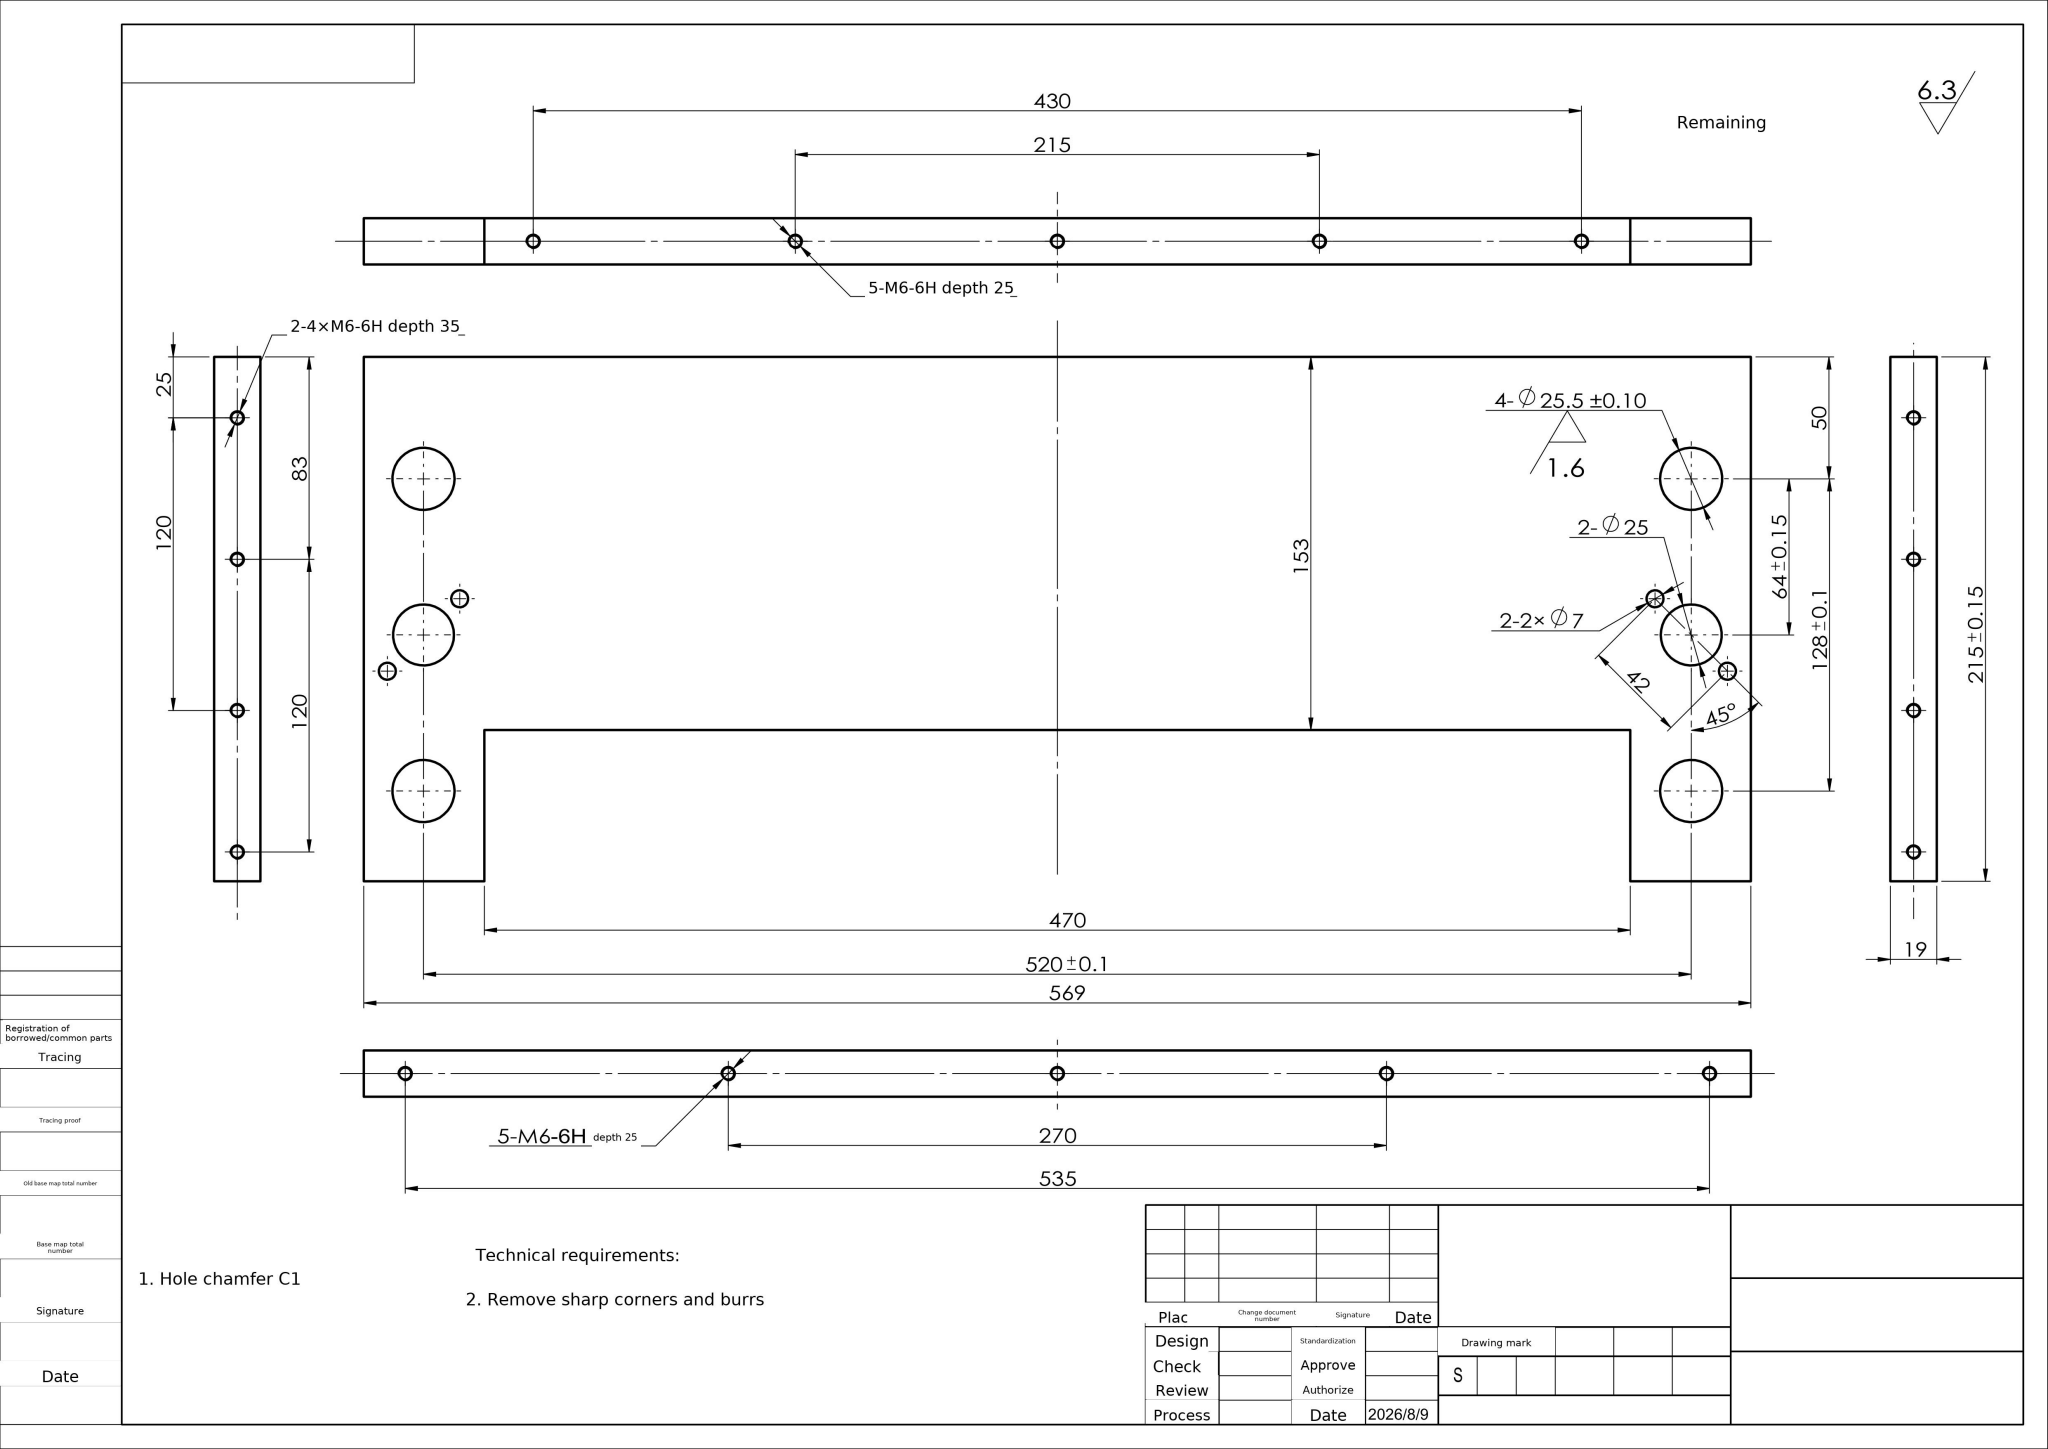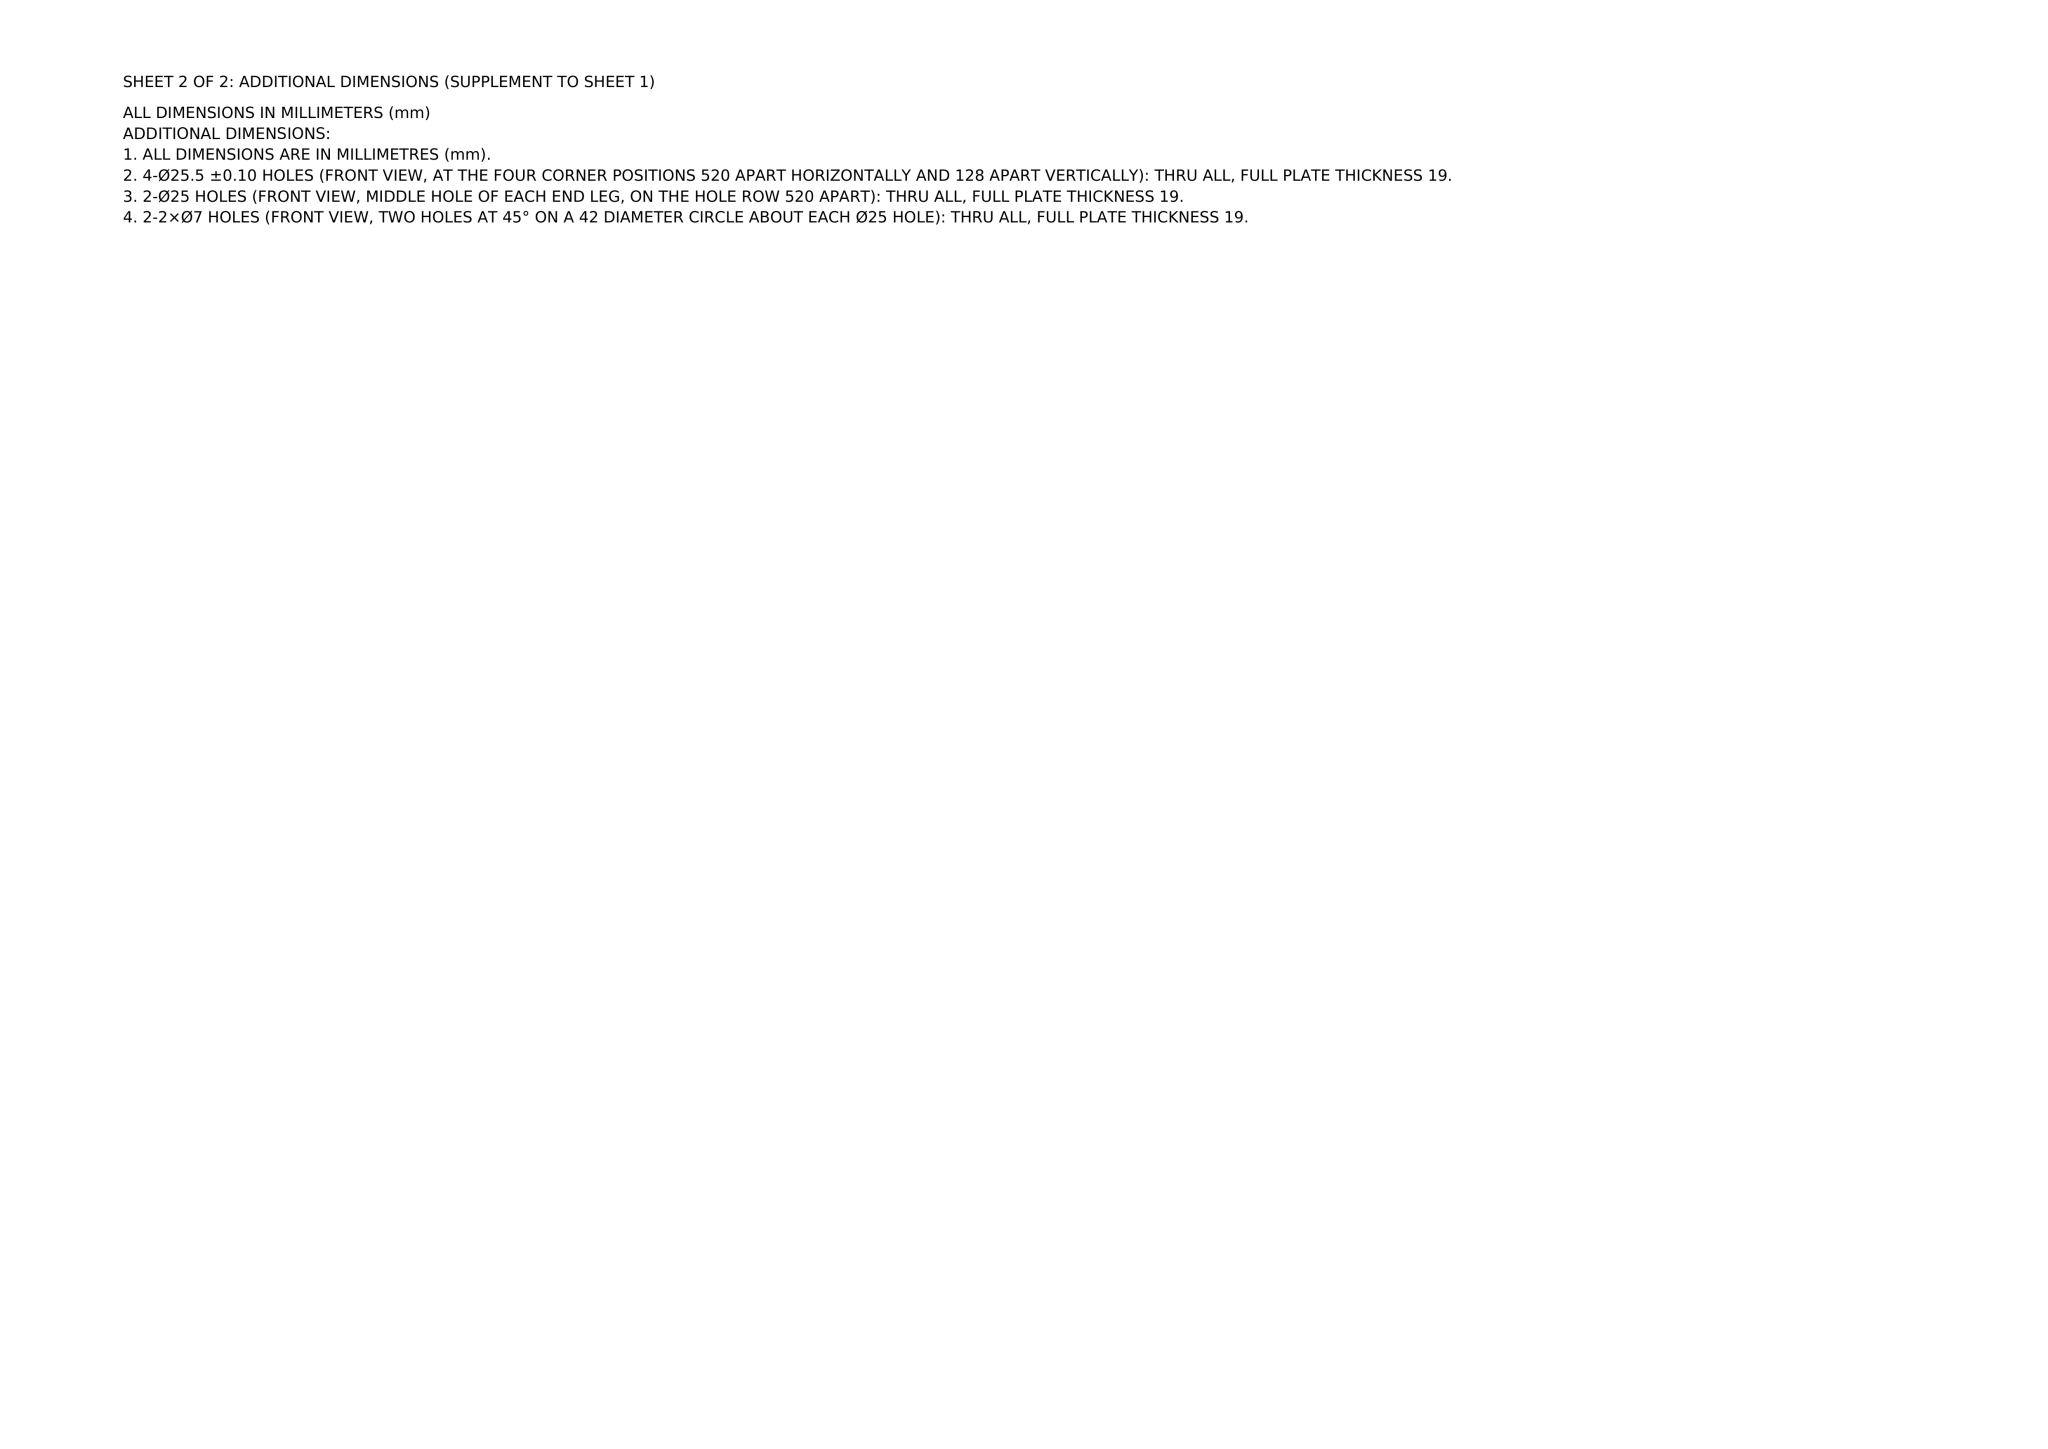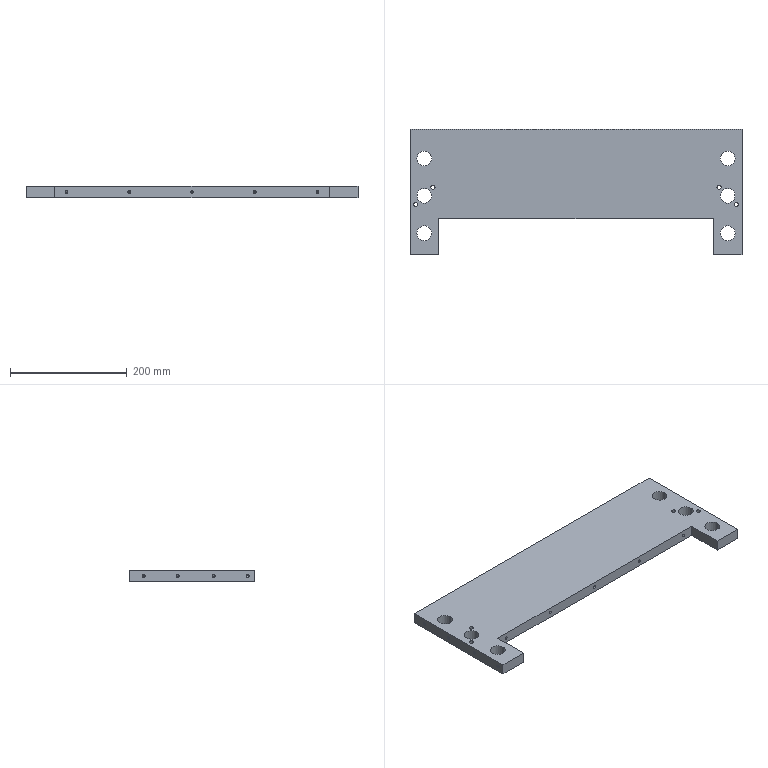Part | NX | mm | U-Shaped Dual-Pedestal Rectangular Mounting Plate | 1 solid | 102 faces | box 569 x 215 x 19 mm | volume 1700790 mm3 | cylinder 56 | cone 36 | plane 10 | commonest cylinder face diameters 5 x36 7 x8 25.5 x8 25 x4